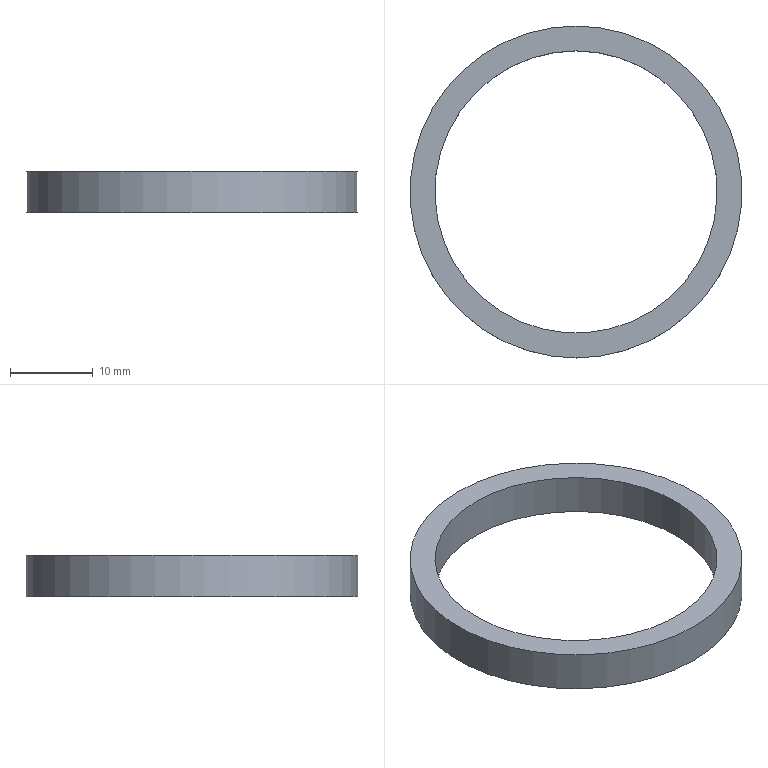Component | NX | PISTON_SEAL | 1 solid | 4 faces | box 40 x 40 x 5 mm | volume 1744 mm3 | cylinder 2 | plane 2 | commonest cylinder face diameters 40 x1 34 x1
STEP:
#1=CARTESIAN_POINT('',(0.,0.,0.));
#2=DIRECTION('',(0.,0.,1.));
#3=DIRECTION('',(1.,0.,0.));
#4=AXIS2_PLACEMENT_3D('',#1,#2,#3);
#5=CARTESIAN_POINT('',(0.,20.,-127.5));
#6=VERTEX_POINT('',#5);
#7=CARTESIAN_POINT('',(0.,0.,-127.5));
#8=DIRECTION('',(0.,0.,1.));
#9=DIRECTION('',(0.,1.,0.));
#10=AXIS2_PLACEMENT_3D('',#7,#8,#9);
#11=CIRCLE('',#10,20.);
#12=CARTESIAN_POINT('',(0.,0.,-127.5));
#13=DIRECTION('',(0.,0.,-1.));
#14=DIRECTION('',(0.,-1.,0.));
#15=AXIS2_PLACEMENT_3D('',#12,#13,#14);
#16=CYLINDRICAL_SURFACE('',#15,20.);
#17=CARTESIAN_POINT('',(9.425,0.));
#18=DIRECTION('',(-1.,0.));
#19=VECTOR('',#18,1.);
#20=LINE('',#17,#19);
#21=(GEOMETRIC_REPRESENTATION_CONTEXT(2)PARAMETRIC_REPRESENTATION_CONTEXT()REPRESENTATION_CONTEXT('',''));
#22=DEFINITIONAL_REPRESENTATION('',(#20),#21);
#23=PCURVE('',#16,#22);
#24=CARTESIAN_POINT('',(0.,0.,-127.5));
#25=DIRECTION('',(0.,0.,1.));
#26=DIRECTION('',(0.,1.,0.));
#27=AXIS2_PLACEMENT_3D('',#24,#25,#26);
#28=PLANE('',#27);
#29=CARTESIAN_POINT('',(0.,0.));
#30=DIRECTION('',(1.,0.));
#31=AXIS2_PLACEMENT_2D('',#29,#30);
#32=CIRCLE('',#31,20.);
#33=(GEOMETRIC_REPRESENTATION_CONTEXT(2)PARAMETRIC_REPRESENTATION_CONTEXT()REPRESENTATION_CONTEXT('',''));
#34=DEFINITIONAL_REPRESENTATION('',(#32),#33);
#35=PCURVE('',#28,#34);
#36=SURFACE_CURVE('',#11,(#23,#35),.PCURVE_S1.);
#37=EDGE_CURVE('',#6,#6,#36,.T.);
#38=ORIENTED_EDGE('',*,*,#37,.F.);
#39=CARTESIAN_POINT('',(0.,20.,-132.5));
#40=VERTEX_POINT('',#39);
#41=CARTESIAN_POINT('',(-0.,20.,-127.5));
#42=CARTESIAN_POINT('',(-0.,20.,-132.5));
#43=B_SPLINE_CURVE_WITH_KNOTS('',1,(#41,#42),.UNSPECIFIED.,.F.,.F.,(2,2),(0.,5.),.PIECEWISE_BEZIER_KNOTS.);
#44=CARTESIAN_POINT('',(9.425,0.));
#45=DIRECTION('',(0.,1.));
#46=VECTOR('',#45,1.);
#47=LINE('',#44,#46);
#48=(GEOMETRIC_REPRESENTATION_CONTEXT(2)PARAMETRIC_REPRESENTATION_CONTEXT()REPRESENTATION_CONTEXT('',''));
#49=DEFINITIONAL_REPRESENTATION('',(#47),#48);
#50=PCURVE('',#16,#49);
#51=CARTESIAN_POINT('',(3.142,0.));
#52=DIRECTION('',(0.,1.));
#53=VECTOR('',#52,1.);
#54=LINE('',#51,#53);
#55=(GEOMETRIC_REPRESENTATION_CONTEXT(2)PARAMETRIC_REPRESENTATION_CONTEXT()REPRESENTATION_CONTEXT('',''));
#56=DEFINITIONAL_REPRESENTATION('',(#54),#55);
#57=PCURVE('',#16,#56);
#58=SEAM_CURVE('',#43,(#50,#57),.PCURVE_S1.);
#59=EDGE_CURVE('',#6,#40,#58,.T.);
#60=ORIENTED_EDGE('',*,*,#59,.T.);
#61=CARTESIAN_POINT('',(0.,0.,-132.5));
#62=DIRECTION('',(0.,0.,1.));
#63=DIRECTION('',(0.,1.,0.));
#64=AXIS2_PLACEMENT_3D('',#61,#62,#63);
#65=CIRCLE('',#64,20.);
#66=CARTESIAN_POINT('',(9.425,5.));
#67=DIRECTION('',(-1.,0.));
#68=VECTOR('',#67,1.);
#69=LINE('',#66,#68);
#70=(GEOMETRIC_REPRESENTATION_CONTEXT(2)PARAMETRIC_REPRESENTATION_CONTEXT()REPRESENTATION_CONTEXT('',''));
#71=DEFINITIONAL_REPRESENTATION('',(#69),#70);
#72=PCURVE('',#16,#71);
#73=CARTESIAN_POINT('',(0.,0.,-132.5));
#74=DIRECTION('',(0.,0.,1.));
#75=DIRECTION('',(0.,1.,0.));
#76=AXIS2_PLACEMENT_3D('',#73,#74,#75);
#77=PLANE('',#76);
#78=CARTESIAN_POINT('',(0.,0.));
#79=DIRECTION('',(1.,0.));
#80=AXIS2_PLACEMENT_2D('',#78,#79);
#81=CIRCLE('',#80,20.);
#82=(GEOMETRIC_REPRESENTATION_CONTEXT(2)PARAMETRIC_REPRESENTATION_CONTEXT()REPRESENTATION_CONTEXT('',''));
#83=DEFINITIONAL_REPRESENTATION('',(#81),#82);
#84=PCURVE('',#77,#83);
#85=SURFACE_CURVE('',#65,(#72,#84),.PCURVE_S1.);
#86=EDGE_CURVE('',#40,#40,#85,.T.);
#87=ORIENTED_EDGE('',*,*,#86,.T.);
#88=ORIENTED_EDGE('',*,*,#59,.F.);
#89=EDGE_LOOP('',(#38,#60,#87,#88));
#90=FACE_BOUND('',#89,.T.);
#91=ADVANCED_FACE('',(#90),#16,.T.);
#92=CARTESIAN_POINT('',(0.,17.,-127.5));
#93=VERTEX_POINT('',#92);
#94=CARTESIAN_POINT('',(0.,0.,-127.5));
#95=DIRECTION('',(0.,0.,1.));
#96=DIRECTION('',(0.,1.,0.));
#97=AXIS2_PLACEMENT_3D('',#94,#95,#96);
#98=CIRCLE('',#97,17.);
#99=CARTESIAN_POINT('',(0.,0.,-127.5));
#100=DIRECTION('',(0.,0.,-1.));
#101=DIRECTION('',(0.,-1.,0.));
#102=AXIS2_PLACEMENT_3D('',#99,#100,#101);
#103=CYLINDRICAL_SURFACE('',#102,17.);
#104=CARTESIAN_POINT('',(9.425,0.));
#105=DIRECTION('',(-1.,0.));
#106=VECTOR('',#105,1.);
#107=LINE('',#104,#106);
#108=(GEOMETRIC_REPRESENTATION_CONTEXT(2)PARAMETRIC_REPRESENTATION_CONTEXT()REPRESENTATION_CONTEXT('',''));
#109=DEFINITIONAL_REPRESENTATION('',(#107),#108);
#110=PCURVE('',#103,#109);
#111=CARTESIAN_POINT('',(0.,0.));
#112=DIRECTION('',(1.,0.));
#113=AXIS2_PLACEMENT_2D('',#111,#112);
#114=CIRCLE('',#113,17.);
#115=(GEOMETRIC_REPRESENTATION_CONTEXT(2)PARAMETRIC_REPRESENTATION_CONTEXT()REPRESENTATION_CONTEXT('',''));
#116=DEFINITIONAL_REPRESENTATION('',(#114),#115);
#117=PCURVE('',#28,#116);
#118=SURFACE_CURVE('',#98,(#110,#117),.PCURVE_S1.);
#119=EDGE_CURVE('',#93,#93,#118,.T.);
#120=ORIENTED_EDGE('',*,*,#119,.F.);
#121=CARTESIAN_POINT('',(0.,17.,-132.5));
#122=VERTEX_POINT('',#121);
#123=CARTESIAN_POINT('',(-0.,17.,-127.5));
#124=CARTESIAN_POINT('',(-0.,17.,-132.5));
#125=B_SPLINE_CURVE_WITH_KNOTS('',1,(#123,#124),.UNSPECIFIED.,.F.,.F.,(2,2),(0.,5.),.PIECEWISE_BEZIER_KNOTS.);
#126=CARTESIAN_POINT('',(9.425,0.));
#127=DIRECTION('',(0.,1.));
#128=VECTOR('',#127,1.);
#129=LINE('',#126,#128);
#130=(GEOMETRIC_REPRESENTATION_CONTEXT(2)PARAMETRIC_REPRESENTATION_CONTEXT()REPRESENTATION_CONTEXT('',''));
#131=DEFINITIONAL_REPRESENTATION('',(#129),#130);
#132=PCURVE('',#103,#131);
#133=CARTESIAN_POINT('',(3.142,0.));
#134=DIRECTION('',(0.,1.));
#135=VECTOR('',#134,1.);
#136=LINE('',#133,#135);
#137=(GEOMETRIC_REPRESENTATION_CONTEXT(2)PARAMETRIC_REPRESENTATION_CONTEXT()REPRESENTATION_CONTEXT('',''));
#138=DEFINITIONAL_REPRESENTATION('',(#136),#137);
#139=PCURVE('',#103,#138);
#140=SEAM_CURVE('',#125,(#132,#139),.PCURVE_S1.);
#141=EDGE_CURVE('',#93,#122,#140,.T.);
#142=ORIENTED_EDGE('',*,*,#141,.T.);
#143=CARTESIAN_POINT('',(0.,0.,-132.5));
#144=DIRECTION('',(0.,0.,1.));
#145=DIRECTION('',(0.,1.,0.));
#146=AXIS2_PLACEMENT_3D('',#143,#144,#145);
#147=CIRCLE('',#146,17.);
#148=CARTESIAN_POINT('',(9.425,5.));
#149=DIRECTION('',(-1.,0.));
#150=VECTOR('',#149,1.);
#151=LINE('',#148,#150);
#152=(GEOMETRIC_REPRESENTATION_CONTEXT(2)PARAMETRIC_REPRESENTATION_CONTEXT()REPRESENTATION_CONTEXT('',''));
#153=DEFINITIONAL_REPRESENTATION('',(#151),#152);
#154=PCURVE('',#103,#153);
#155=CARTESIAN_POINT('',(0.,0.));
#156=DIRECTION('',(1.,0.));
#157=AXIS2_PLACEMENT_2D('',#155,#156);
#158=CIRCLE('',#157,17.);
#159=(GEOMETRIC_REPRESENTATION_CONTEXT(2)PARAMETRIC_REPRESENTATION_CONTEXT()REPRESENTATION_CONTEXT('',''));
#160=DEFINITIONAL_REPRESENTATION('',(#158),#159);
#161=PCURVE('',#77,#160);
#162=SURFACE_CURVE('',#147,(#154,#161),.PCURVE_S1.);
#163=EDGE_CURVE('',#122,#122,#162,.T.);
#164=ORIENTED_EDGE('',*,*,#163,.T.);
#165=ORIENTED_EDGE('',*,*,#141,.F.);
#166=EDGE_LOOP('',(#120,#142,#164,#165));
#167=FACE_BOUND('',#166,.F.);
#168=ADVANCED_FACE('',(#167),#103,.F.);
#169=ORIENTED_EDGE('',*,*,#37,.T.);
#170=EDGE_LOOP('',(#169));
#171=FACE_BOUND('',#170,.T.);
#172=ORIENTED_EDGE('',*,*,#119,.F.);
#173=EDGE_LOOP('',(#172));
#174=FACE_BOUND('',#173,.T.);
#175=ADVANCED_FACE('',(#171,#174),#28,.T.);
#176=ORIENTED_EDGE('',*,*,#86,.F.);
#177=EDGE_LOOP('',(#176));
#178=FACE_BOUND('',#177,.T.);
#179=ORIENTED_EDGE('',*,*,#163,.T.);
#180=EDGE_LOOP('',(#179));
#181=FACE_BOUND('',#180,.T.);
#182=ADVANCED_FACE('',(#178,#181),#77,.F.);
#183=CLOSED_SHELL('',(#91,#168,#175,#182));
#184=MANIFOLD_SOLID_BREP('',#183);
#185=(LENGTH_UNIT()NAMED_UNIT(*)SI_UNIT(.MILLI.,.METRE.));
#186=UNCERTAINTY_MEASURE_WITH_UNIT(LENGTH_MEASURE(0.00001),#185,'','');
#187=(NAMED_UNIT(*)PLANE_ANGLE_UNIT()SI_UNIT($,.RADIAN.));
#188=(NAMED_UNIT(*)SI_UNIT($,.STERADIAN.)SOLID_ANGLE_UNIT());
#189=(GEOMETRIC_REPRESENTATION_CONTEXT(3)GLOBAL_UNCERTAINTY_ASSIGNED_CONTEXT((#186))GLOBAL_UNIT_ASSIGNED_CONTEXT((#185,#187,#188))REPRESENTATION_CONTEXT('',''));
#190=ADVANCED_BREP_SHAPE_REPRESENTATION('',(#4,#184),#189);